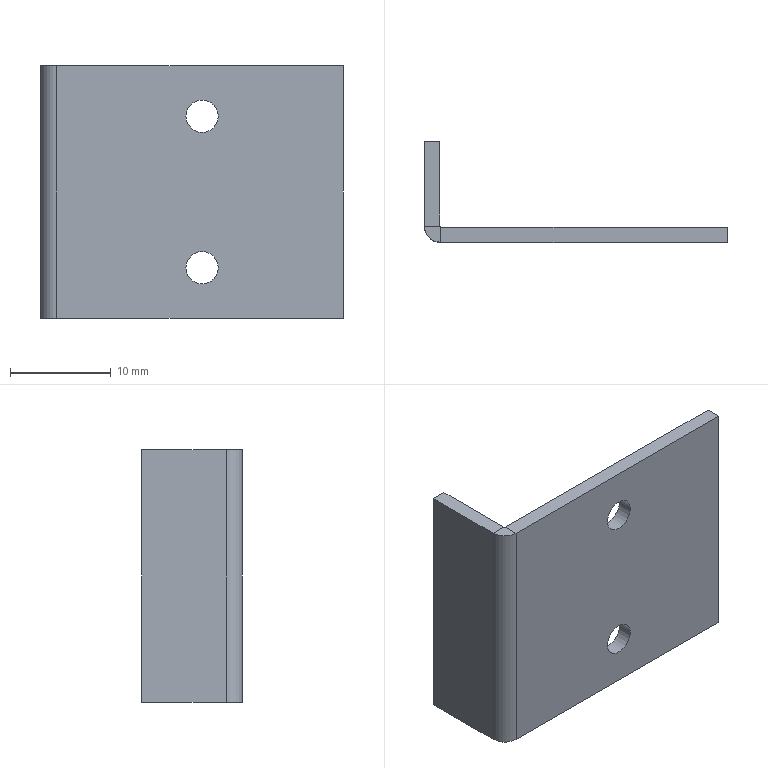Component | SolidWorks | Lampshade-1_Lampshade5-1 | 1 solid | 18 faces | volume 1406 mm3 | plane 12 | cylinder 6 | commonest cylinder face diameters 3.2 x5 0.2 x1